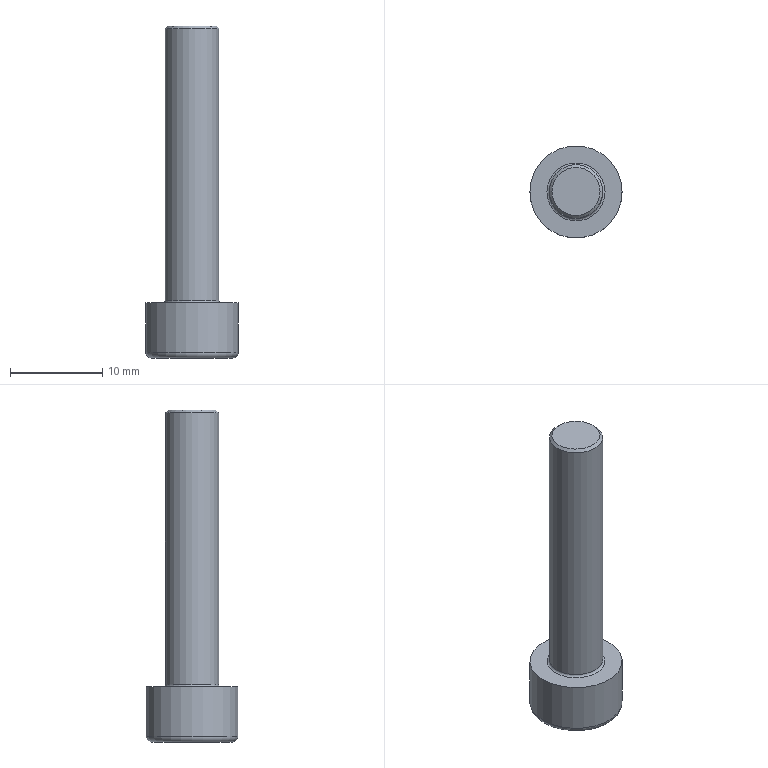Component | NX | SCREW_M6X30 | 1 solid | 27 faces | volume 1169 mm3 | plane 15 | cone 8 | cylinder 2 | torus 2 | commonest cylinder face diameters 5.795 x1 10 x1